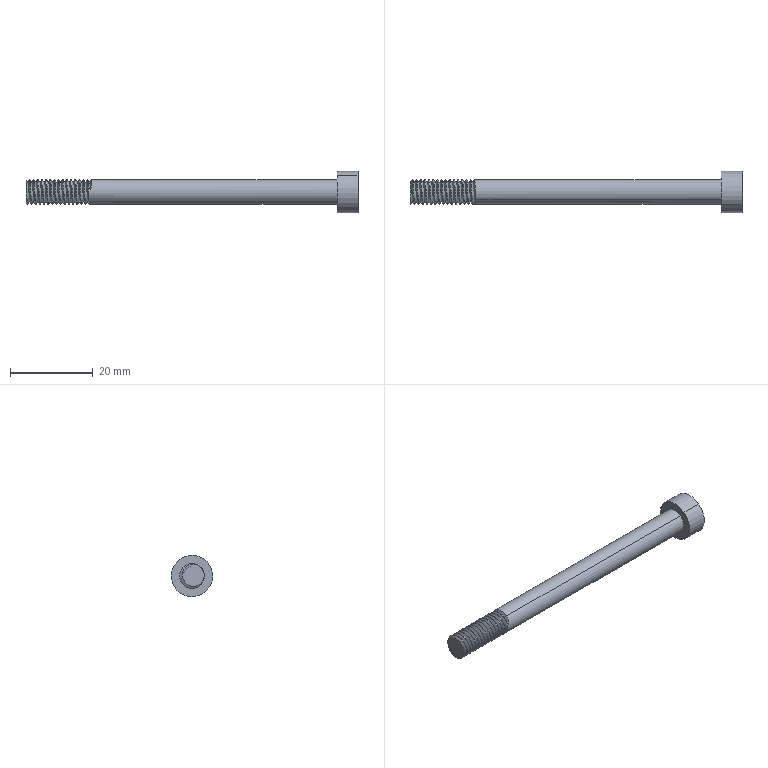Component | SolidWorks | OuterBagSealingGuideRod-2 | 1 solid | 41 faces | volume 2420 mm3 | cylinder 34 | plane 5 | spline 2 | commonest cylinder face diameters 6 x32 10 x2